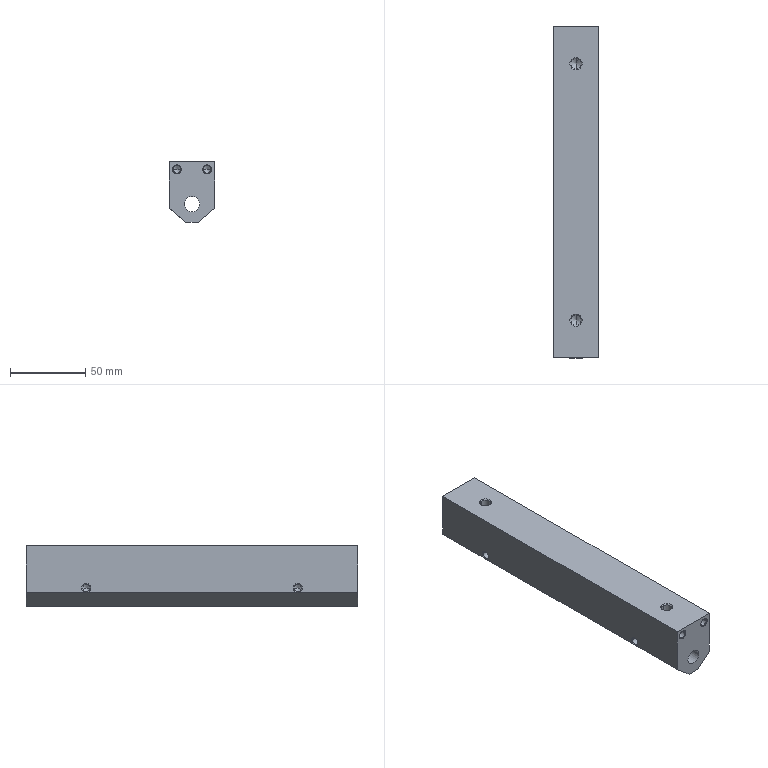Component | SolidWorks | DirectPressureVerticalSeal-1_VerticalSealRoller-1 | 1 solid | 62 faces | volume 220799 mm3 | cone 32 | cylinder 22 | plane 8 | commonest cylinder face diameters 5 x16 6.8 x4 10.2 x2